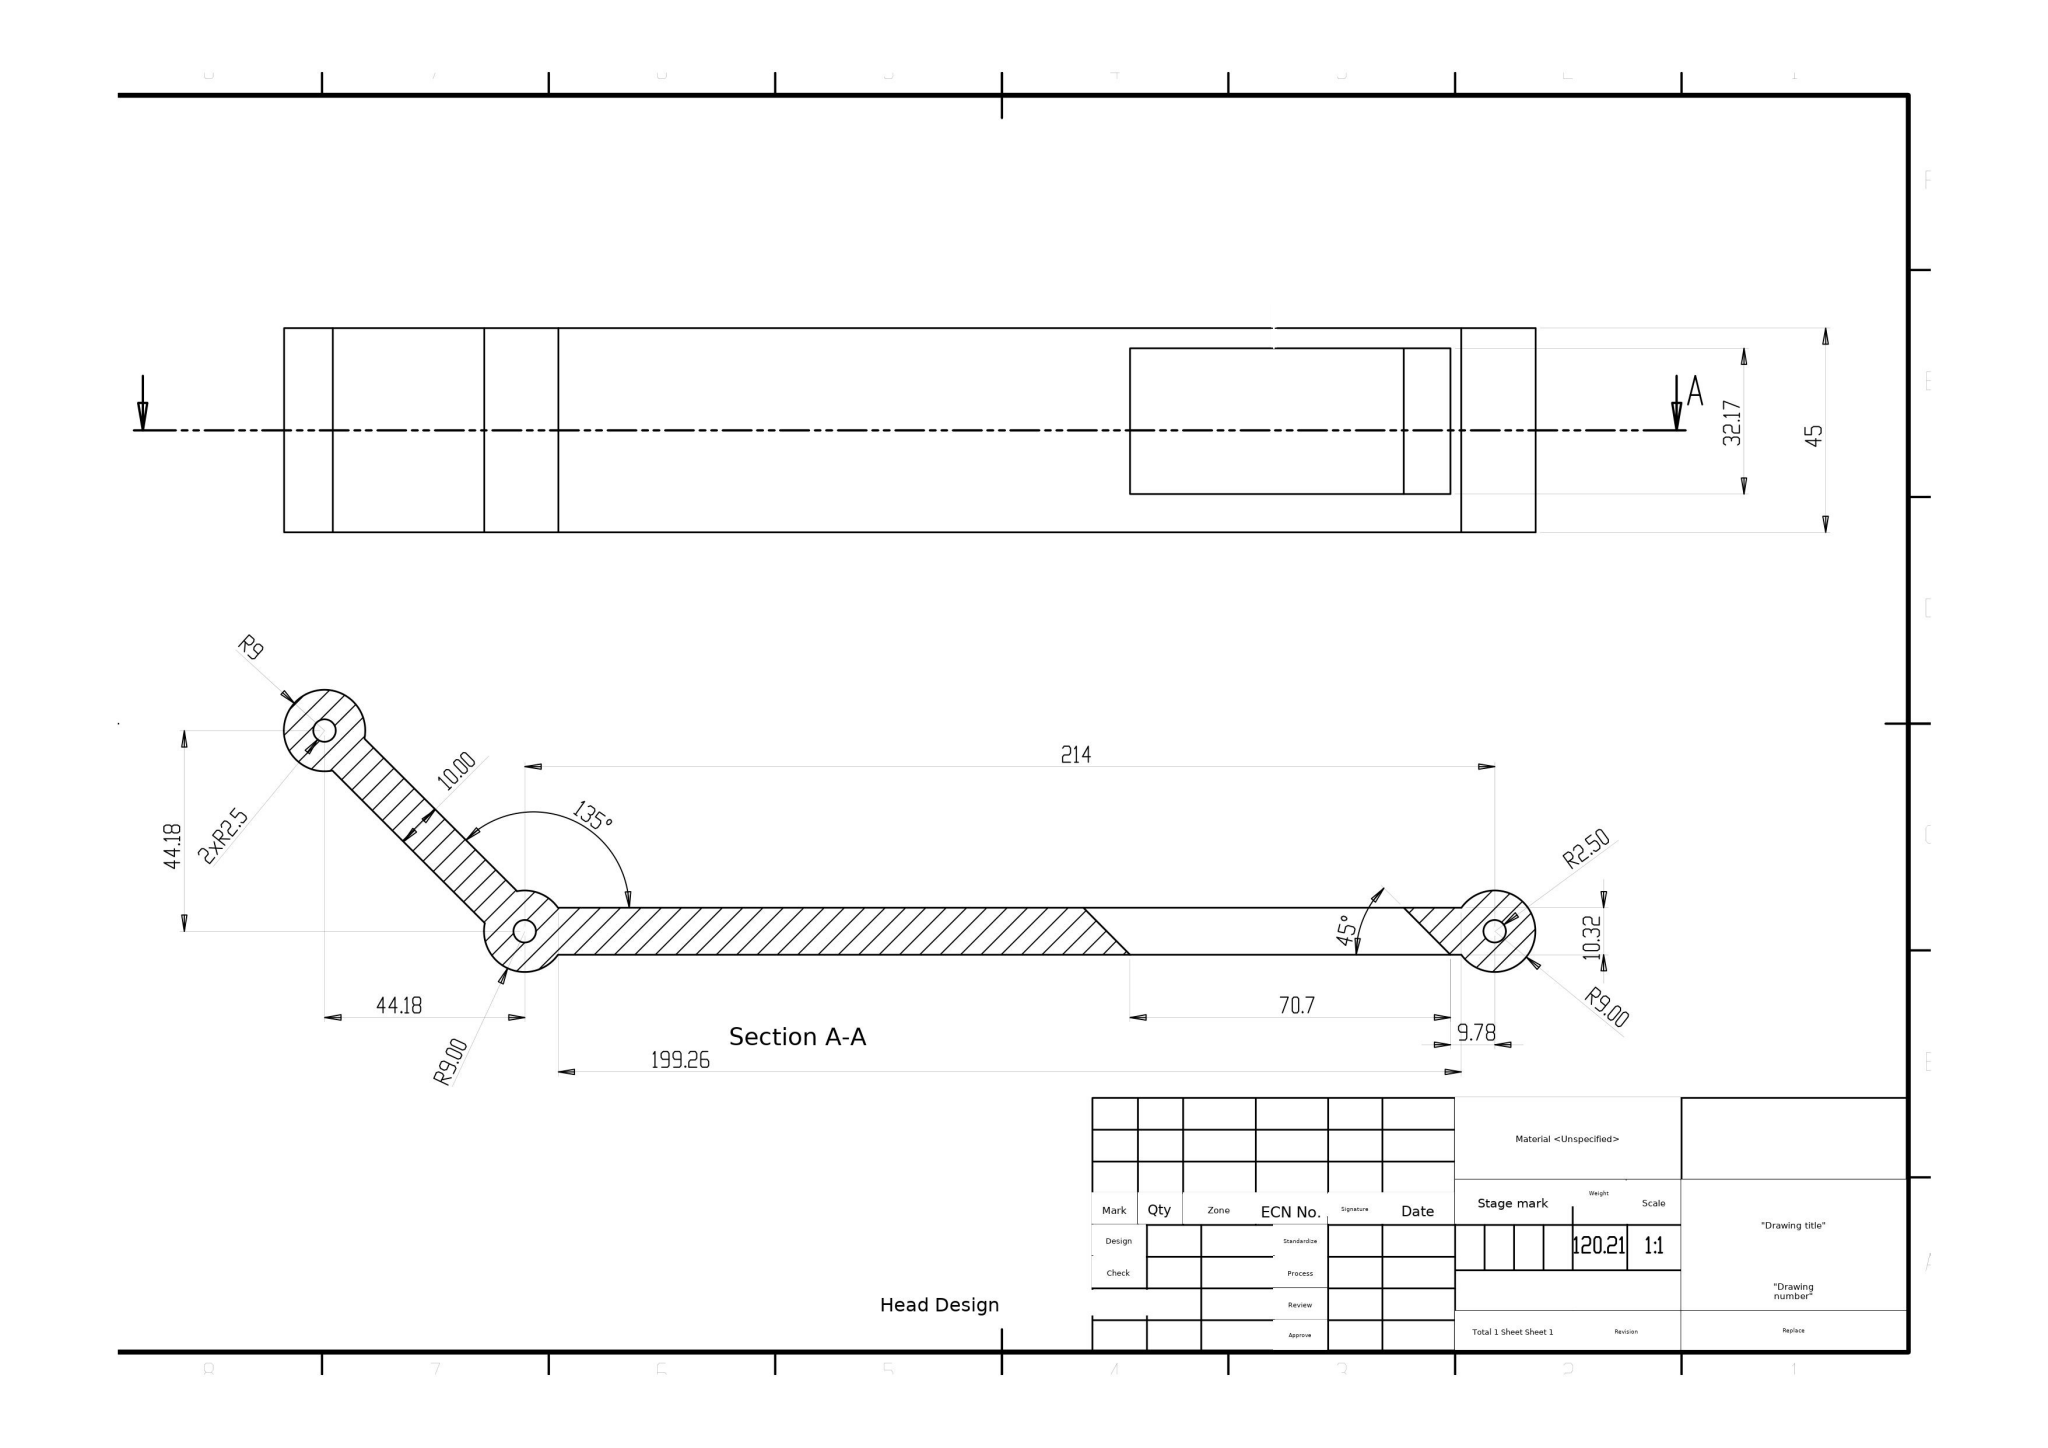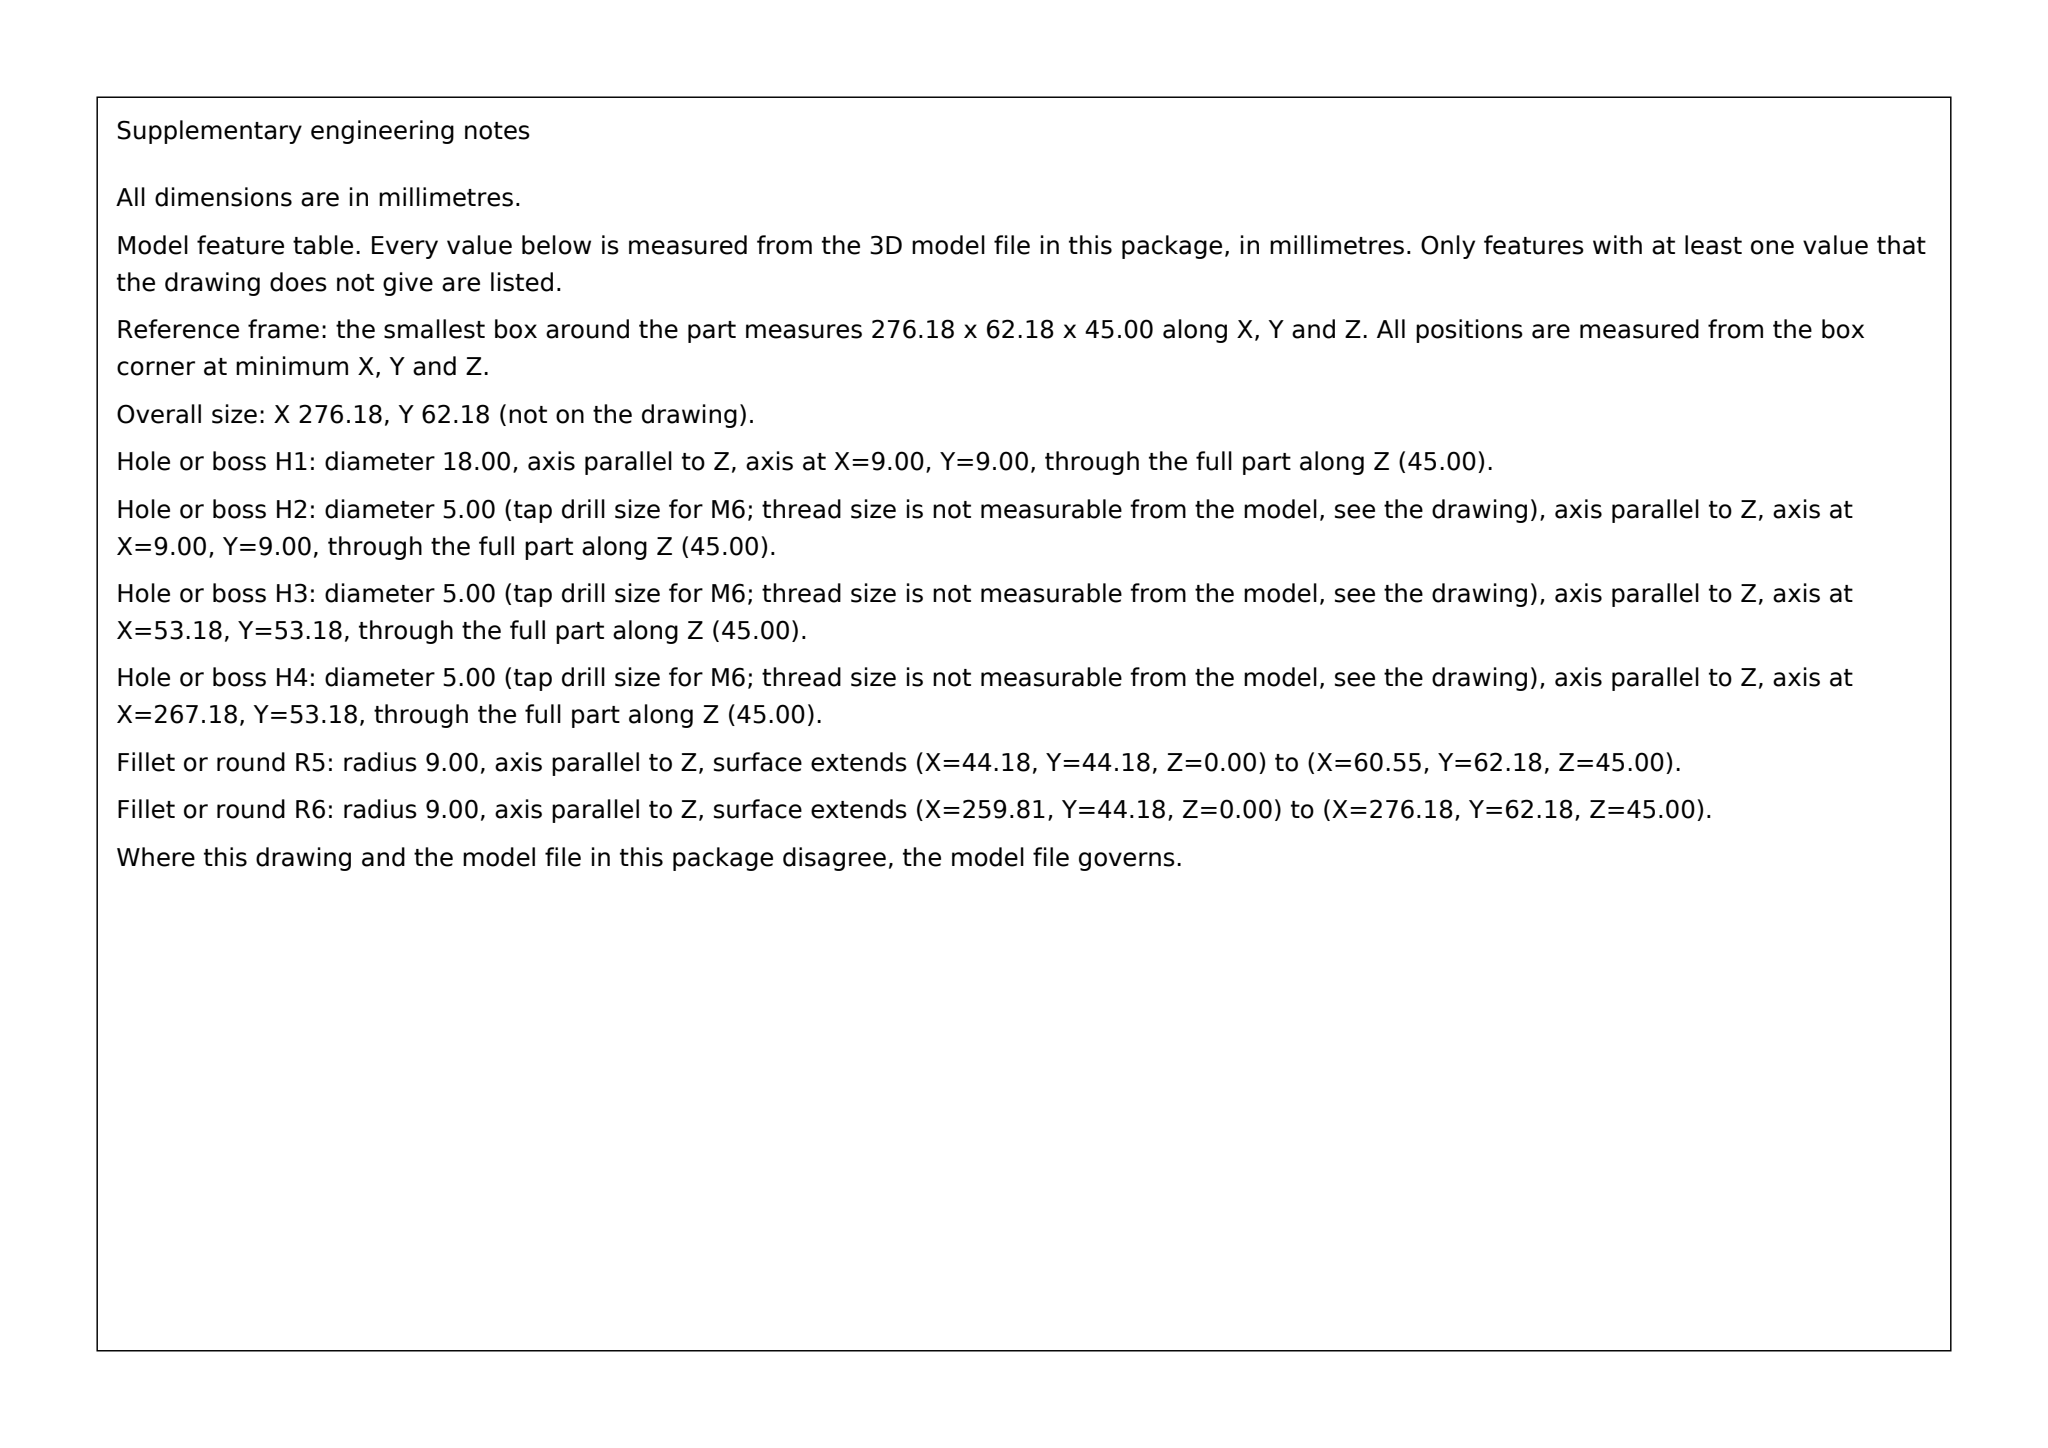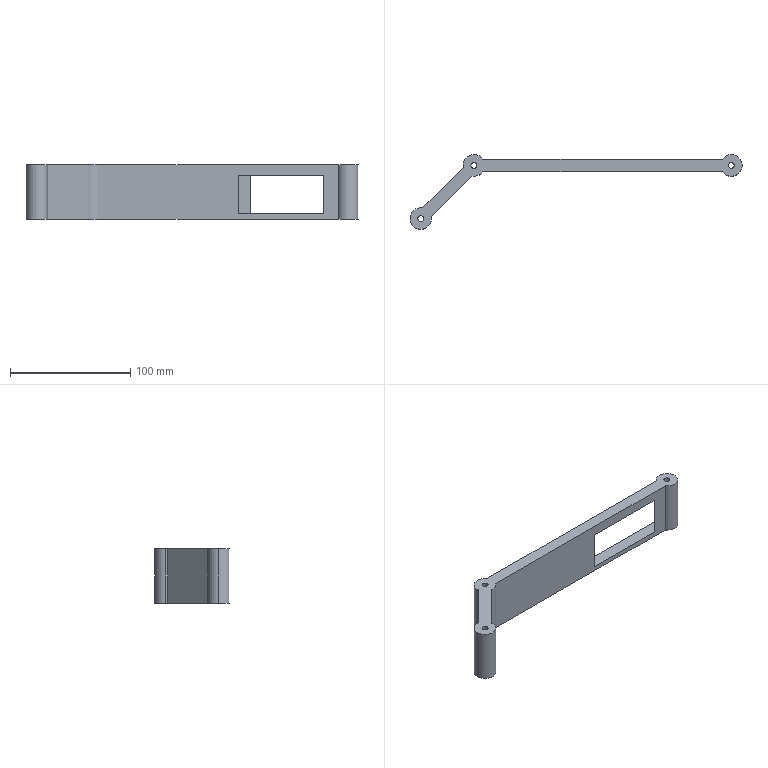Part | SolidWorks | mm | 1 solid | 23 faces | box 276.18 x 62.18 x 45 mm | volume 120214 mm3 | cylinder 13 | plane 10 | commonest cylinder face diameters 18 x7 5 x6
STEP:
#1=CARTESIAN_POINT('',(123.185,-5.162,36.594));
#2=VERTEX_POINT('',#1);
#3=CARTESIAN_POINT('',(133.509,5.162,36.594));
#4=VERTEX_POINT('',#3);
#5=CARTESIAN_POINT('',(10.993,-117.357,36.594));
#6=DIRECTION('',(0.7071,0.7071,0.));
#7=VECTOR('',#6,1000.);
#8=LINE('',#5,#7);
#9=EDGE_CURVE('',#2,#4,#8,.T.);
#10=ORIENTED_EDGE('',*,*,#9,.T.);
#11=CARTESIAN_POINT('',(204.219,5.162,36.594));
#12=VERTEX_POINT('',#11);
#13=CARTESIAN_POINT('',(-0.,5.162,36.594));
#14=DIRECTION('',(-1.,-0.,0.));
#15=VECTOR('',#14,1000.);
#16=LINE('',#13,#15);
#17=EDGE_CURVE('',#12,#4,#16,.T.);
#18=ORIENTED_EDGE('',*,*,#17,.F.);
#19=CARTESIAN_POINT('',(193.895,-5.162,36.594));
#20=VERTEX_POINT('',#19);
#21=CARTESIAN_POINT('',(46.349,-152.711,36.594));
#22=DIRECTION('',(0.7071,0.7071,0.));
#23=VECTOR('',#22,1000.);
#24=LINE('',#21,#23);
#25=EDGE_CURVE('',#20,#12,#24,.T.);
#26=ORIENTED_EDGE('',*,*,#25,.F.);
#27=CARTESIAN_POINT('',(-0.,-5.162,36.594));
#28=DIRECTION('',(1.,0.,-0.));
#29=VECTOR('',#28,1000.);
#30=LINE('',#27,#29);
#31=EDGE_CURVE('',#2,#20,#30,.T.);
#32=ORIENTED_EDGE('',*,*,#31,.F.);
#33=EDGE_LOOP('',(#10,#18,#26,#32));
#34=FACE_OUTER_BOUND('',#33,.T.);
#35=CARTESIAN_POINT('',(10.993,-117.357,36.594));
#36=DIRECTION('',(-0.,0.,-1.));
#37=DIRECTION('',(-1.,0.,0.));
#38=AXIS2_PLACEMENT_3D('',#35,#36,#37);
#39=PLANE('',#38);
#40=ADVANCED_FACE('',(#34),#39,.T.);
#41=ORIENTED_EDGE('',*,*,#25,.T.);
#42=CARTESIAN_POINT('',(204.219,5.162,4.421));
#43=VERTEX_POINT('',#42);
#44=CARTESIAN_POINT('',(204.219,5.162,45.));
#45=DIRECTION('',(0.,0.,1.));
#46=VECTOR('',#45,1000.);
#47=LINE('',#44,#46);
#48=EDGE_CURVE('',#43,#12,#47,.T.);
#49=ORIENTED_EDGE('',*,*,#48,.F.);
#50=CARTESIAN_POINT('',(193.895,-5.162,4.421));
#51=VERTEX_POINT('',#50);
#52=CARTESIAN_POINT('',(46.349,-152.711,4.421));
#53=DIRECTION('',(0.7071,0.7071,0.));
#54=VECTOR('',#53,1000.);
#55=LINE('',#52,#54);
#56=EDGE_CURVE('',#51,#43,#55,.T.);
#57=ORIENTED_EDGE('',*,*,#56,.F.);
#58=CARTESIAN_POINT('',(193.895,-5.162,45.));
#59=DIRECTION('',(-0.,0.,-1.));
#60=VECTOR('',#59,1000.);
#61=LINE('',#58,#60);
#62=EDGE_CURVE('',#20,#51,#61,.T.);
#63=ORIENTED_EDGE('',*,*,#62,.F.);
#64=EDGE_LOOP('',(#41,#49,#57,#63));
#65=FACE_OUTER_BOUND('',#64,.T.);
#66=CARTESIAN_POINT('',(46.349,-152.711,36.594));
#67=DIRECTION('',(-0.7071,0.7071,0.));
#68=DIRECTION('',(0.,0.,1.));
#69=AXIS2_PLACEMENT_3D('',#66,#67,#68);
#70=PLANE('',#69);
#71=ADVANCED_FACE('',(#65),#70,.T.);
#72=ORIENTED_EDGE('',*,*,#56,.T.);
#73=CARTESIAN_POINT('',(133.509,5.162,4.421));
#74=VERTEX_POINT('',#73);
#75=CARTESIAN_POINT('',(-0.,5.162,4.421));
#76=DIRECTION('',(1.,0.,-0.));
#77=VECTOR('',#76,1000.);
#78=LINE('',#75,#77);
#79=EDGE_CURVE('',#74,#43,#78,.T.);
#80=ORIENTED_EDGE('',*,*,#79,.F.);
#81=CARTESIAN_POINT('',(123.185,-5.162,4.421));
#82=VERTEX_POINT('',#81);
#83=CARTESIAN_POINT('',(10.993,-117.357,4.421));
#84=DIRECTION('',(0.7071,0.7071,0.));
#85=VECTOR('',#84,1000.);
#86=LINE('',#83,#85);
#87=EDGE_CURVE('',#82,#74,#86,.T.);
#88=ORIENTED_EDGE('',*,*,#87,.F.);
#89=CARTESIAN_POINT('',(-0.,-5.162,4.421));
#90=DIRECTION('',(-1.,0.,0.));
#91=VECTOR('',#90,1000.);
#92=LINE('',#89,#91);
#93=EDGE_CURVE('',#51,#82,#92,.T.);
#94=ORIENTED_EDGE('',*,*,#93,.F.);
#95=EDGE_LOOP('',(#72,#80,#88,#94));
#96=FACE_OUTER_BOUND('',#95,.T.);
#97=CARTESIAN_POINT('',(46.349,-152.711,4.421));
#98=DIRECTION('',(0.,-0.,1.));
#99=DIRECTION('',(0.,-1.,-0.));
#100=AXIS2_PLACEMENT_3D('',#97,#98,#99);
#101=PLANE('',#100);
#102=ADVANCED_FACE('',(#96),#101,.T.);
#103=ORIENTED_EDGE('',*,*,#87,.T.);
#104=CARTESIAN_POINT('',(133.509,5.162,45.));
#105=DIRECTION('',(-0.,-0.,-1.));
#106=VECTOR('',#105,1000.);
#107=LINE('',#104,#106);
#108=EDGE_CURVE('',#4,#74,#107,.T.);
#109=ORIENTED_EDGE('',*,*,#108,.F.);
#110=ORIENTED_EDGE('',*,*,#9,.F.);
#111=CARTESIAN_POINT('',(123.185,-5.162,45.));
#112=DIRECTION('',(0.,0.,1.));
#113=VECTOR('',#112,1000.);
#114=LINE('',#111,#113);
#115=EDGE_CURVE('',#82,#2,#114,.T.);
#116=ORIENTED_EDGE('',*,*,#115,.F.);
#117=EDGE_LOOP('',(#103,#109,#110,#116));
#118=FACE_OUTER_BOUND('',#117,.T.);
#119=CARTESIAN_POINT('',(10.993,-117.357,4.421));
#120=DIRECTION('',(0.7071,-0.7071,-0.));
#121=DIRECTION('',(0.,0.,-1.));
#122=AXIS2_PLACEMENT_3D('',#119,#120,#121);
#123=PLANE('',#122);
#124=ADVANCED_FACE('',(#118),#123,.T.);
#125=CARTESIAN_POINT('',(-46.682,-44.182,0.));
#126=VERTEX_POINT('',#125);
#127=CARTESIAN_POINT('',(-41.682,-44.182,0.));
#128=VERTEX_POINT('',#127);
#129=CARTESIAN_POINT('',(-44.182,-44.182,0.));
#130=DIRECTION('',(0.,0.,1.));
#131=DIRECTION('',(1.,0.,0.));
#132=AXIS2_PLACEMENT_3D('',#129,#130,#131);
#133=CIRCLE('',#132,2.5);
#134=EDGE_CURVE('',#126,#128,#133,.T.);
#135=ORIENTED_EDGE('',*,*,#134,.T.);
#136=CARTESIAN_POINT('',(-44.182,-44.182,0.));
#137=DIRECTION('',(0.,0.,1.));
#138=DIRECTION('',(1.,0.,0.));
#139=AXIS2_PLACEMENT_3D('',#136,#137,#138);
#140=CIRCLE('',#139,2.5);
#141=EDGE_CURVE('',#128,#126,#140,.T.);
#142=ORIENTED_EDGE('',*,*,#141,.T.);
#143=EDGE_LOOP('',(#135,#142));
#144=FACE_BOUND('',#143,.T.);
#145=CARTESIAN_POINT('',(211.5,0.,0.));
#146=VERTEX_POINT('',#145);
#147=CARTESIAN_POINT('',(216.5,0.,0.));
#148=VERTEX_POINT('',#147);
#149=CARTESIAN_POINT('',(214.,0.,0.));
#150=DIRECTION('',(0.,0.,1.));
#151=DIRECTION('',(1.,0.,0.));
#152=AXIS2_PLACEMENT_3D('',#149,#150,#151);
#153=CIRCLE('',#152,2.5);
#154=EDGE_CURVE('',#146,#148,#153,.T.);
#155=ORIENTED_EDGE('',*,*,#154,.T.);
#156=CARTESIAN_POINT('',(214.,0.,0.));
#157=DIRECTION('',(0.,0.,1.));
#158=DIRECTION('',(1.,0.,0.));
#159=AXIS2_PLACEMENT_3D('',#156,#157,#158);
#160=CIRCLE('',#159,2.5);
#161=EDGE_CURVE('',#148,#146,#160,.T.);
#162=ORIENTED_EDGE('',*,*,#161,.T.);
#163=EDGE_LOOP('',(#155,#162));
#164=FACE_BOUND('',#163,.T.);
#165=CARTESIAN_POINT('',(-2.5,0.,0.));
#166=VERTEX_POINT('',#165);
#167=CARTESIAN_POINT('',(2.5,0.,0.));
#168=VERTEX_POINT('',#167);
#169=CARTESIAN_POINT('',(0.,0.,0.));
#170=DIRECTION('',(0.,0.,1.));
#171=DIRECTION('',(1.,0.,0.));
#172=AXIS2_PLACEMENT_3D('',#169,#170,#171);
#173=CIRCLE('',#172,2.5);
#174=EDGE_CURVE('',#166,#168,#173,.T.);
#175=ORIENTED_EDGE('',*,*,#174,.T.);
#176=CARTESIAN_POINT('',(0.,0.,0.));
#177=DIRECTION('',(0.,0.,1.));
#178=DIRECTION('',(1.,0.,0.));
#179=AXIS2_PLACEMENT_3D('',#176,#177,#178);
#180=CIRCLE('',#179,2.5);
#181=EDGE_CURVE('',#168,#166,#180,.T.);
#182=ORIENTED_EDGE('',*,*,#181,.T.);
#183=EDGE_LOOP('',(#175,#182));
#184=FACE_BOUND('',#183,.T.);
#185=CARTESIAN_POINT('',(7.372,5.162,0.));
#186=VERTEX_POINT('',#185);
#187=CARTESIAN_POINT('',(-9.,0.,0.));
#188=VERTEX_POINT('',#187);
#189=CARTESIAN_POINT('',(0.,0.,0.));
#190=DIRECTION('',(0.,0.,1.));
#191=DIRECTION('',(1.,0.,0.));
#192=AXIS2_PLACEMENT_3D('',#189,#190,#191);
#193=CIRCLE('',#192,9.);
#194=EDGE_CURVE('',#186,#188,#193,.T.);
#195=ORIENTED_EDGE('',*,*,#194,.F.);
#196=CARTESIAN_POINT('',(206.628,5.162,0.));
#197=VERTEX_POINT('',#196);
#198=CARTESIAN_POINT('',(-0.,5.162,0.));
#199=DIRECTION('',(1.,0.,0.));
#200=VECTOR('',#199,1000.);
#201=LINE('',#198,#200);
#202=EDGE_CURVE('',#186,#197,#201,.T.);
#203=ORIENTED_EDGE('',*,*,#202,.T.);
#204=CARTESIAN_POINT('',(206.628,-5.162,0.));
#205=VERTEX_POINT('',#204);
#206=CARTESIAN_POINT('',(214.,0.,0.));
#207=DIRECTION('',(0.,0.,1.));
#208=DIRECTION('',(1.,0.,0.));
#209=AXIS2_PLACEMENT_3D('',#206,#207,#208);
#210=CIRCLE('',#209,9.);
#211=EDGE_CURVE('',#205,#197,#210,.T.);
#212=ORIENTED_EDGE('',*,*,#211,.F.);
#213=CARTESIAN_POINT('',(7.372,-5.162,0.));
#214=VERTEX_POINT('',#213);
#215=CARTESIAN_POINT('',(0.,-5.162,0.));
#216=DIRECTION('',(-1.,0.,0.));
#217=VECTOR('',#216,1000.);
#218=LINE('',#215,#217);
#219=EDGE_CURVE('',#205,#214,#218,.T.);
#220=ORIENTED_EDGE('',*,*,#219,.T.);
#221=CARTESIAN_POINT('',(-1.756,-8.827,0.));
#222=VERTEX_POINT('',#221);
#223=CARTESIAN_POINT('',(0.,0.,0.));
#224=DIRECTION('',(0.,0.,1.));
#225=DIRECTION('',(1.,0.,0.));
#226=AXIS2_PLACEMENT_3D('',#223,#224,#225);
#227=CIRCLE('',#226,9.);
#228=EDGE_CURVE('',#222,#214,#227,.T.);
#229=ORIENTED_EDGE('',*,*,#228,.F.);
#230=CARTESIAN_POINT('',(-35.355,-42.426,0.));
#231=VERTEX_POINT('',#230);
#232=CARTESIAN_POINT('',(3.536,-3.536,0.));
#233=DIRECTION('',(-0.7071,-0.7071,0.));
#234=VECTOR('',#233,1000.);
#235=LINE('',#232,#234);
#236=EDGE_CURVE('',#222,#231,#235,.T.);
#237=ORIENTED_EDGE('',*,*,#236,.T.);
#238=CARTESIAN_POINT('',(-35.182,-44.182,0.));
#239=VERTEX_POINT('',#238);
#240=CARTESIAN_POINT('',(-44.182,-44.182,0.));
#241=DIRECTION('',(0.,0.,1.));
#242=DIRECTION('',(1.,0.,0.));
#243=AXIS2_PLACEMENT_3D('',#240,#241,#242);
#244=CIRCLE('',#243,9.);
#245=EDGE_CURVE('',#239,#231,#244,.T.);
#246=ORIENTED_EDGE('',*,*,#245,.F.);
#247=CARTESIAN_POINT('',(-53.182,-44.182,0.));
#248=VERTEX_POINT('',#247);
#249=CARTESIAN_POINT('',(-44.182,-44.182,0.));
#250=DIRECTION('',(0.,0.,1.));
#251=DIRECTION('',(1.,0.,0.));
#252=AXIS2_PLACEMENT_3D('',#249,#250,#251);
#253=CIRCLE('',#252,9.);
#254=EDGE_CURVE('',#248,#239,#253,.T.);
#255=ORIENTED_EDGE('',*,*,#254,.F.);
#256=CARTESIAN_POINT('',(-42.426,-35.355,0.));
#257=VERTEX_POINT('',#256);
#258=CARTESIAN_POINT('',(-44.182,-44.182,0.));
#259=DIRECTION('',(0.,0.,1.));
#260=DIRECTION('',(1.,0.,0.));
#261=AXIS2_PLACEMENT_3D('',#258,#259,#260);
#262=CIRCLE('',#261,9.);
#263=EDGE_CURVE('',#257,#248,#262,.T.);
#264=ORIENTED_EDGE('',*,*,#263,.F.);
#265=CARTESIAN_POINT('',(-8.827,-1.756,0.));
#266=VERTEX_POINT('',#265);
#267=CARTESIAN_POINT('',(-3.536,3.536,0.));
#268=DIRECTION('',(-0.7071,-0.7071,0.));
#269=VECTOR('',#268,1000.);
#270=LINE('',#267,#269);
#271=EDGE_CURVE('',#266,#257,#270,.T.);
#272=ORIENTED_EDGE('',*,*,#271,.F.);
#273=CARTESIAN_POINT('',(0.,0.,0.));
#274=DIRECTION('',(0.,0.,1.));
#275=DIRECTION('',(1.,0.,0.));
#276=AXIS2_PLACEMENT_3D('',#273,#274,#275);
#277=CIRCLE('',#276,9.);
#278=EDGE_CURVE('',#188,#266,#277,.T.);
#279=ORIENTED_EDGE('',*,*,#278,.F.);
#280=EDGE_LOOP('',(#195,#203,#212,#220,#229,#237,#246,#255,#264,#272,#279));
#281=FACE_OUTER_BOUND('',#280,.T.);
#282=CARTESIAN_POINT('',(0.,0.,0.));
#283=DIRECTION('',(0.,0.,1.));
#284=DIRECTION('',(1.,0.,0.));
#285=AXIS2_PLACEMENT_3D('',#282,#283,#284);
#286=PLANE('',#285);
#287=ADVANCED_FACE('',(#144,#164,#184,#281),#286,.F.);
#288=CARTESIAN_POINT('',(-46.682,-44.182,45.));
#289=VERTEX_POINT('',#288);
#290=CARTESIAN_POINT('',(-41.682,-44.182,45.));
#291=VERTEX_POINT('',#290);
#292=CARTESIAN_POINT('',(-44.182,-44.182,45.));
#293=DIRECTION('',(0.,0.,1.));
#294=DIRECTION('',(1.,0.,0.));
#295=AXIS2_PLACEMENT_3D('',#292,#293,#294);
#296=CIRCLE('',#295,2.5);
#297=EDGE_CURVE('',#289,#291,#296,.T.);
#298=ORIENTED_EDGE('',*,*,#297,.F.);
#299=CARTESIAN_POINT('',(-44.182,-44.182,45.));
#300=DIRECTION('',(0.,0.,1.));
#301=DIRECTION('',(1.,0.,0.));
#302=AXIS2_PLACEMENT_3D('',#299,#300,#301);
#303=CIRCLE('',#302,2.5);
#304=EDGE_CURVE('',#291,#289,#303,.T.);
#305=ORIENTED_EDGE('',*,*,#304,.F.);
#306=EDGE_LOOP('',(#298,#305));
#307=FACE_BOUND('',#306,.T.);
#308=CARTESIAN_POINT('',(211.5,0.,45.));
#309=VERTEX_POINT('',#308);
#310=CARTESIAN_POINT('',(216.5,0.,45.));
#311=VERTEX_POINT('',#310);
#312=CARTESIAN_POINT('',(214.,0.,45.));
#313=DIRECTION('',(0.,0.,1.));
#314=DIRECTION('',(1.,0.,0.));
#315=AXIS2_PLACEMENT_3D('',#312,#313,#314);
#316=CIRCLE('',#315,2.5);
#317=EDGE_CURVE('',#309,#311,#316,.T.);
#318=ORIENTED_EDGE('',*,*,#317,.F.);
#319=CARTESIAN_POINT('',(214.,0.,45.));
#320=DIRECTION('',(0.,0.,1.));
#321=DIRECTION('',(1.,0.,0.));
#322=AXIS2_PLACEMENT_3D('',#319,#320,#321);
#323=CIRCLE('',#322,2.5);
#324=EDGE_CURVE('',#311,#309,#323,.T.);
#325=ORIENTED_EDGE('',*,*,#324,.F.);
#326=EDGE_LOOP('',(#318,#325));
#327=FACE_BOUND('',#326,.T.);
#328=CARTESIAN_POINT('',(-2.5,0.,45.));
#329=VERTEX_POINT('',#328);
#330=CARTESIAN_POINT('',(2.5,0.,45.));
#331=VERTEX_POINT('',#330);
#332=CARTESIAN_POINT('',(0.,0.,45.));
#333=DIRECTION('',(0.,0.,1.));
#334=DIRECTION('',(1.,0.,0.));
#335=AXIS2_PLACEMENT_3D('',#332,#333,#334);
#336=CIRCLE('',#335,2.5);
#337=EDGE_CURVE('',#329,#331,#336,.T.);
#338=ORIENTED_EDGE('',*,*,#337,.F.);
#339=CARTESIAN_POINT('',(0.,0.,45.));
#340=DIRECTION('',(0.,0.,1.));
#341=DIRECTION('',(1.,0.,0.));
#342=AXIS2_PLACEMENT_3D('',#339,#340,#341);
#343=CIRCLE('',#342,2.5);
#344=EDGE_CURVE('',#331,#329,#343,.T.);
#345=ORIENTED_EDGE('',*,*,#344,.F.);
#346=EDGE_LOOP('',(#338,#345));
#347=FACE_BOUND('',#346,.T.);
#348=CARTESIAN_POINT('',(7.372,5.162,45.));
#349=VERTEX_POINT('',#348);
#350=CARTESIAN_POINT('',(-9.,0.,45.));
#351=VERTEX_POINT('',#350);
#352=CARTESIAN_POINT('',(0.,0.,45.));
#353=DIRECTION('',(0.,0.,1.));
#354=DIRECTION('',(1.,0.,0.));
#355=AXIS2_PLACEMENT_3D('',#352,#353,#354);
#356=CIRCLE('',#355,9.);
#357=EDGE_CURVE('',#349,#351,#356,.T.);
#358=ORIENTED_EDGE('',*,*,#357,.T.);
#359=CARTESIAN_POINT('',(-8.827,-1.756,45.));
#360=VERTEX_POINT('',#359);
#361=CARTESIAN_POINT('',(0.,0.,45.));
#362=DIRECTION('',(0.,0.,1.));
#363=DIRECTION('',(1.,0.,0.));
#364=AXIS2_PLACEMENT_3D('',#361,#362,#363);
#365=CIRCLE('',#364,9.);
#366=EDGE_CURVE('',#351,#360,#365,.T.);
#367=ORIENTED_EDGE('',*,*,#366,.T.);
#368=CARTESIAN_POINT('',(-42.426,-35.355,45.));
#369=VERTEX_POINT('',#368);
#370=CARTESIAN_POINT('',(-3.536,3.536,45.));
#371=DIRECTION('',(-0.7071,-0.7071,0.));
#372=VECTOR('',#371,1000.);
#373=LINE('',#370,#372);
#374=EDGE_CURVE('',#360,#369,#373,.T.);
#375=ORIENTED_EDGE('',*,*,#374,.T.);
#376=CARTESIAN_POINT('',(-53.182,-44.182,45.));
#377=VERTEX_POINT('',#376);
#378=CARTESIAN_POINT('',(-44.182,-44.182,45.));
#379=DIRECTION('',(0.,0.,1.));
#380=DIRECTION('',(1.,0.,0.));
#381=AXIS2_PLACEMENT_3D('',#378,#379,#380);
#382=CIRCLE('',#381,9.);
#383=EDGE_CURVE('',#369,#377,#382,.T.);
#384=ORIENTED_EDGE('',*,*,#383,.T.);
#385=CARTESIAN_POINT('',(-35.182,-44.182,45.));
#386=VERTEX_POINT('',#385);
#387=CARTESIAN_POINT('',(-44.182,-44.182,45.));
#388=DIRECTION('',(0.,0.,1.));
#389=DIRECTION('',(1.,0.,0.));
#390=AXIS2_PLACEMENT_3D('',#387,#388,#389);
#391=CIRCLE('',#390,9.);
#392=EDGE_CURVE('',#377,#386,#391,.T.);
#393=ORIENTED_EDGE('',*,*,#392,.T.);
#394=CARTESIAN_POINT('',(-35.355,-42.426,45.));
#395=VERTEX_POINT('',#394);
#396=CARTESIAN_POINT('',(-44.182,-44.182,45.));
#397=DIRECTION('',(0.,0.,1.));
#398=DIRECTION('',(1.,0.,0.));
#399=AXIS2_PLACEMENT_3D('',#396,#397,#398);
#400=CIRCLE('',#399,9.);
#401=EDGE_CURVE('',#386,#395,#400,.T.);
#402=ORIENTED_EDGE('',*,*,#401,.T.);
#403=CARTESIAN_POINT('',(-1.756,-8.827,45.));
#404=VERTEX_POINT('',#403);
#405=CARTESIAN_POINT('',(3.536,-3.536,45.));
#406=DIRECTION('',(-0.7071,-0.7071,0.));
#407=VECTOR('',#406,1000.);
#408=LINE('',#405,#407);
#409=EDGE_CURVE('',#404,#395,#408,.T.);
#410=ORIENTED_EDGE('',*,*,#409,.F.);
#411=CARTESIAN_POINT('',(7.372,-5.162,45.));
#412=VERTEX_POINT('',#411);
#413=CARTESIAN_POINT('',(0.,0.,45.));
#414=DIRECTION('',(0.,0.,1.));
#415=DIRECTION('',(1.,0.,0.));
#416=AXIS2_PLACEMENT_3D('',#413,#414,#415);
#417=CIRCLE('',#416,9.);
#418=EDGE_CURVE('',#404,#412,#417,.T.);
#419=ORIENTED_EDGE('',*,*,#418,.T.);
#420=CARTESIAN_POINT('',(206.628,-5.162,45.));
#421=VERTEX_POINT('',#420);
#422=CARTESIAN_POINT('',(0.,-5.162,45.));
#423=DIRECTION('',(-1.,0.,0.));
#424=VECTOR('',#423,1000.);
#425=LINE('',#422,#424);
#426=EDGE_CURVE('',#421,#412,#425,.T.);
#427=ORIENTED_EDGE('',*,*,#426,.F.);
#428=CARTESIAN_POINT('',(206.628,5.162,45.));
#429=VERTEX_POINT('',#428);
#430=CARTESIAN_POINT('',(214.,0.,45.));
#431=DIRECTION('',(0.,0.,1.));
#432=DIRECTION('',(1.,0.,0.));
#433=AXIS2_PLACEMENT_3D('',#430,#431,#432);
#434=CIRCLE('',#433,9.);
#435=EDGE_CURVE('',#421,#429,#434,.T.);
#436=ORIENTED_EDGE('',*,*,#435,.T.);
#437=CARTESIAN_POINT('',(-0.,5.162,45.));
#438=DIRECTION('',(1.,0.,0.));
#439=VECTOR('',#438,1000.);
#440=LINE('',#437,#439);
#441=EDGE_CURVE('',#349,#429,#440,.T.);
#442=ORIENTED_EDGE('',*,*,#441,.F.);
#443=EDGE_LOOP('',(#358,#367,#375,#384,#393,#402,#410,#419,#427,#436,#442));
#444=FACE_OUTER_BOUND('',#443,.T.);
#445=CARTESIAN_POINT('',(0.,0.,45.));
#446=DIRECTION('',(0.,0.,1.));
#447=DIRECTION('',(1.,0.,0.));
#448=AXIS2_PLACEMENT_3D('',#445,#446,#447);
#449=PLANE('',#448);
#450=ADVANCED_FACE('',(#307,#327,#347,#444),#449,.T.);
#451=CARTESIAN_POINT('',(-41.682,-44.182,45.));
#452=DIRECTION('',(0.,0.,-1.));
#453=VECTOR('',#452,1000.);
#454=LINE('',#451,#453);
#455=EDGE_CURVE('',#291,#128,#454,.T.);
#456=ORIENTED_EDGE('',*,*,#455,.F.);
#457=ORIENTED_EDGE('',*,*,#304,.T.);
#458=CARTESIAN_POINT('',(-46.682,-44.182,45.));
#459=DIRECTION('',(0.,0.,-1.));
#460=VECTOR('',#459,1000.);
#461=LINE('',#458,#460);
#462=EDGE_CURVE('',#289,#126,#461,.T.);
#463=ORIENTED_EDGE('',*,*,#462,.T.);
#464=ORIENTED_EDGE('',*,*,#141,.F.);
#465=EDGE_LOOP('',(#456,#457,#463,#464));
#466=FACE_OUTER_BOUND('',#465,.T.);
#467=CARTESIAN_POINT('',(-44.182,-44.182,45.));
#468=DIRECTION('',(0.,0.,-1.));
#469=DIRECTION('',(-1.,0.,0.));
#470=AXIS2_PLACEMENT_3D('',#467,#468,#469);
#471=CYLINDRICAL_SURFACE('',#470,2.5);
#472=ADVANCED_FACE('',(#466),#471,.F.);
#473=CARTESIAN_POINT('',(2.5,0.,45.));
#474=DIRECTION('',(0.,0.,-1.));
#475=VECTOR('',#474,1000.);
#476=LINE('',#473,#475);
#477=EDGE_CURVE('',#331,#168,#476,.T.);
#478=ORIENTED_EDGE('',*,*,#477,.F.);
#479=ORIENTED_EDGE('',*,*,#344,.T.);
#480=CARTESIAN_POINT('',(-2.5,0.,45.));
#481=DIRECTION('',(0.,0.,-1.));
#482=VECTOR('',#481,1000.);
#483=LINE('',#480,#482);
#484=EDGE_CURVE('',#329,#166,#483,.T.);
#485=ORIENTED_EDGE('',*,*,#484,.T.);
#486=ORIENTED_EDGE('',*,*,#181,.F.);
#487=EDGE_LOOP('',(#478,#479,#485,#486));
#488=FACE_OUTER_BOUND('',#487,.T.);
#489=CARTESIAN_POINT('',(0.,0.,45.));
#490=DIRECTION('',(0.,0.,-1.));
#491=DIRECTION('',(-1.,0.,0.));
#492=AXIS2_PLACEMENT_3D('',#489,#490,#491);
#493=CYLINDRICAL_SURFACE('',#492,2.5);
#494=ADVANCED_FACE('',(#488),#493,.F.);
#495=CARTESIAN_POINT('',(216.5,0.,45.));
#496=DIRECTION('',(0.,0.,-1.));
#497=VECTOR('',#496,1000.);
#498=LINE('',#495,#497);
#499=EDGE_CURVE('',#311,#148,#498,.T.);
#500=ORIENTED_EDGE('',*,*,#499,.F.);
#501=ORIENTED_EDGE('',*,*,#324,.T.);
#502=CARTESIAN_POINT('',(211.5,0.,45.));
#503=DIRECTION('',(0.,0.,-1.));
#504=VECTOR('',#503,1000.);
#505=LINE('',#502,#504);
#506=EDGE_CURVE('',#309,#146,#505,.T.);
#507=ORIENTED_EDGE('',*,*,#506,.T.);
#508=ORIENTED_EDGE('',*,*,#161,.F.);
#509=EDGE_LOOP('',(#500,#501,#507,#508));
#510=FACE_OUTER_BOUND('',#509,.T.);
#511=CARTESIAN_POINT('',(214.,0.,45.));
#512=DIRECTION('',(0.,0.,-1.));
#513=DIRECTION('',(-1.,0.,0.));
#514=AXIS2_PLACEMENT_3D('',#511,#512,#513);
#515=CYLINDRICAL_SURFACE('',#514,2.5);
#516=ADVANCED_FACE('',(#510),#515,.F.);
#517=ORIENTED_EDGE('',*,*,#211,.T.);
#518=CARTESIAN_POINT('',(206.628,5.162,45.));
#519=DIRECTION('',(0.,0.,-1.));
#520=VECTOR('',#519,1000.);
#521=LINE('',#518,#520);
#522=EDGE_CURVE('',#429,#197,#521,.T.);
#523=ORIENTED_EDGE('',*,*,#522,.F.);
#524=ORIENTED_EDGE('',*,*,#435,.F.);
#525=CARTESIAN_POINT('',(206.628,-5.162,45.));
#526=DIRECTION('',(0.,0.,-1.));
#527=VECTOR('',#526,1000.);
#528=LINE('',#525,#527);
#529=EDGE_CURVE('',#421,#205,#528,.T.);
#530=ORIENTED_EDGE('',*,*,#529,.T.);
#531=EDGE_LOOP('',(#517,#523,#524,#530));
#532=FACE_OUTER_BOUND('',#531,.T.);
#533=CARTESIAN_POINT('',(214.,0.,45.));
#534=DIRECTION('',(0.,0.,-1.));
#535=DIRECTION('',(-1.,0.,0.));
#536=AXIS2_PLACEMENT_3D('',#533,#534,#535);
#537=CYLINDRICAL_SURFACE('',#536,9.);
#538=ADVANCED_FACE('',(#532),#537,.T.);
#539=ORIENTED_EDGE('',*,*,#228,.T.);
#540=CARTESIAN_POINT('',(7.372,-5.162,45.));
#541=DIRECTION('',(0.,0.,-1.));
#542=VECTOR('',#541,1000.);
#543=LINE('',#540,#542);
#544=EDGE_CURVE('',#412,#214,#543,.T.);
#545=ORIENTED_EDGE('',*,*,#544,.F.);
#546=ORIENTED_EDGE('',*,*,#418,.F.);
#547=CARTESIAN_POINT('',(-1.756,-8.827,45.));
#548=DIRECTION('',(0.,0.,-1.));
#549=VECTOR('',#548,1000.);
#550=LINE('',#547,#549);
#551=EDGE_CURVE('',#404,#222,#550,.T.);
#552=ORIENTED_EDGE('',*,*,#551,.T.);
#553=EDGE_LOOP('',(#539,#545,#546,#552));
#554=FACE_OUTER_BOUND('',#553,.T.);
#555=CARTESIAN_POINT('',(0.,0.,45.));
#556=DIRECTION('',(0.,0.,-1.));
#557=DIRECTION('',(-1.,0.,0.));
#558=AXIS2_PLACEMENT_3D('',#555,#556,#557);
#559=CYLINDRICAL_SURFACE('',#558,9.);
#560=ADVANCED_FACE('',(#554),#559,.T.);
#561=ORIENTED_EDGE('',*,*,#236,.F.);
#562=ORIENTED_EDGE('',*,*,#551,.F.);
#563=ORIENTED_EDGE('',*,*,#409,.T.);
#564=CARTESIAN_POINT('',(-35.355,-42.426,45.));
#565=DIRECTION('',(0.,0.,-1.));
#566=VECTOR('',#565,1000.);
#567=LINE('',#564,#566);
#568=EDGE_CURVE('',#395,#231,#567,.T.);
#569=ORIENTED_EDGE('',*,*,#568,.T.);
#570=EDGE_LOOP('',(#561,#562,#563,#569));
#571=FACE_OUTER_BOUND('',#570,.T.);
#572=CARTESIAN_POINT('',(3.536,-3.536,45.));
#573=DIRECTION('',(0.7071,-0.7071,0.));
#574=DIRECTION('',(0.,0.,-1.));
#575=AXIS2_PLACEMENT_3D('',#572,#573,#574);
#576=PLANE('',#575);
#577=ADVANCED_FACE('',(#571),#576,.T.);
#578=CARTESIAN_POINT('',(-53.182,-44.182,45.));
#579=DIRECTION('',(0.,0.,-1.));
#580=VECTOR('',#579,1000.);
#581=LINE('',#578,#580);
#582=EDGE_CURVE('',#377,#248,#581,.T.);
#583=ORIENTED_EDGE('',*,*,#582,.F.);
#584=ORIENTED_EDGE('',*,*,#383,.F.);
#585=CARTESIAN_POINT('',(-42.426,-35.355,45.));
#586=DIRECTION('',(0.,0.,-1.));
#587=VECTOR('',#586,1000.);
#588=LINE('',#585,#587);
#589=EDGE_CURVE('',#369,#257,#588,.T.);
#590=ORIENTED_EDGE('',*,*,#589,.T.);
#591=ORIENTED_EDGE('',*,*,#263,.T.);
#592=EDGE_LOOP('',(#583,#584,#590,#591));
#593=FACE_OUTER_BOUND('',#592,.T.);
#594=CARTESIAN_POINT('',(-44.182,-44.182,45.));
#595=DIRECTION('',(0.,0.,-1.));
#596=DIRECTION('',(-1.,0.,0.));
#597=AXIS2_PLACEMENT_3D('',#594,#595,#596);
#598=CYLINDRICAL_SURFACE('',#597,9.);
#599=ADVANCED_FACE('',(#593),#598,.T.);
#600=ORIENTED_EDGE('',*,*,#271,.T.);
#601=ORIENTED_EDGE('',*,*,#589,.F.);
#602=ORIENTED_EDGE('',*,*,#374,.F.);
#603=CARTESIAN_POINT('',(-8.827,-1.756,45.));
#604=DIRECTION('',(0.,0.,-1.));
#605=VECTOR('',#604,1000.);
#606=LINE('',#603,#605);
#607=EDGE_CURVE('',#360,#266,#606,.T.);
#608=ORIENTED_EDGE('',*,*,#607,.T.);
#609=EDGE_LOOP('',(#600,#601,#602,#608));
#610=FACE_OUTER_BOUND('',#609,.T.);
#611=CARTESIAN_POINT('',(-3.536,3.536,45.));
#612=DIRECTION('',(0.7071,-0.7071,0.));
#613=DIRECTION('',(0.,0.,-1.));
#614=AXIS2_PLACEMENT_3D('',#611,#612,#613);
#615=PLANE('',#614);
#616=ADVANCED_FACE('',(#610),#615,.F.);
#617=CARTESIAN_POINT('',(-9.,0.,45.));
#618=DIRECTION('',(0.,0.,-1.));
#619=VECTOR('',#618,1000.);
#620=LINE('',#617,#619);
#621=EDGE_CURVE('',#351,#188,#620,.T.);
#622=ORIENTED_EDGE('',*,*,#621,.F.);
#623=ORIENTED_EDGE('',*,*,#357,.F.);
#624=CARTESIAN_POINT('',(7.372,5.162,45.));
#625=DIRECTION('',(0.,0.,-1.));
#626=VECTOR('',#625,1000.);
#627=LINE('',#624,#626);
#628=EDGE_CURVE('',#349,#186,#627,.T.);
#629=ORIENTED_EDGE('',*,*,#628,.T.);
#630=ORIENTED_EDGE('',*,*,#194,.T.);
#631=EDGE_LOOP('',(#622,#623,#629,#630));
#632=FACE_OUTER_BOUND('',#631,.T.);
#633=CARTESIAN_POINT('',(0.,0.,45.));
#634=DIRECTION('',(0.,0.,-1.));
#635=DIRECTION('',(-1.,0.,0.));
#636=AXIS2_PLACEMENT_3D('',#633,#634,#635);
#637=CYLINDRICAL_SURFACE('',#636,9.);
#638=ADVANCED_FACE('',(#632),#637,.T.);
#639=ORIENTED_EDGE('',*,*,#17,.T.);
#640=ORIENTED_EDGE('',*,*,#108,.T.);
#641=ORIENTED_EDGE('',*,*,#79,.T.);
#642=ORIENTED_EDGE('',*,*,#48,.T.);
#643=EDGE_LOOP('',(#639,#640,#641,#642));
#644=FACE_BOUND('',#643,.T.);
#645=ORIENTED_EDGE('',*,*,#202,.F.);
#646=ORIENTED_EDGE('',*,*,#628,.F.);
#647=ORIENTED_EDGE('',*,*,#441,.T.);
#648=ORIENTED_EDGE('',*,*,#522,.T.);
#649=EDGE_LOOP('',(#645,#646,#647,#648));
#650=FACE_OUTER_BOUND('',#649,.T.);
#651=CARTESIAN_POINT('',(-0.,5.162,45.));
#652=DIRECTION('',(-0.,1.,0.));
#653=DIRECTION('',(1.,0.,0.));
#654=AXIS2_PLACEMENT_3D('',#651,#652,#653);
#655=PLANE('',#654);
#656=ADVANCED_FACE('',(#644,#650),#655,.T.);
#657=ORIENTED_EDGE('',*,*,#93,.T.);
#658=ORIENTED_EDGE('',*,*,#115,.T.);
#659=ORIENTED_EDGE('',*,*,#31,.T.);
#660=ORIENTED_EDGE('',*,*,#62,.T.);
#661=EDGE_LOOP('',(#657,#658,#659,#660));
#662=FACE_BOUND('',#661,.T.);
#663=ORIENTED_EDGE('',*,*,#219,.F.);
#664=ORIENTED_EDGE('',*,*,#529,.F.);
#665=ORIENTED_EDGE('',*,*,#426,.T.);
#666=ORIENTED_EDGE('',*,*,#544,.T.);
#667=EDGE_LOOP('',(#663,#664,#665,#666));
#668=FACE_OUTER_BOUND('',#667,.T.);
#669=CARTESIAN_POINT('',(0.,-5.162,45.));
#670=DIRECTION('',(0.,-1.,0.));
#671=DIRECTION('',(0.,0.,-1.));
#672=AXIS2_PLACEMENT_3D('',#669,#670,#671);
#673=PLANE('',#672);
#674=ADVANCED_FACE('',(#662,#668),#673,.T.);
#675=ORIENTED_EDGE('',*,*,#366,.F.);
#676=ORIENTED_EDGE('',*,*,#621,.T.);
#677=ORIENTED_EDGE('',*,*,#278,.T.);
#678=ORIENTED_EDGE('',*,*,#607,.F.);
#679=EDGE_LOOP('',(#675,#676,#677,#678));
#680=FACE_OUTER_BOUND('',#679,.T.);
#681=CARTESIAN_POINT('',(0.,0.,45.));
#682=DIRECTION('',(0.,0.,-1.));
#683=DIRECTION('',(-1.,0.,0.));
#684=AXIS2_PLACEMENT_3D('',#681,#682,#683);
#685=CYLINDRICAL_SURFACE('',#684,9.);
#686=ADVANCED_FACE('',(#680),#685,.T.);
#687=CARTESIAN_POINT('',(-35.182,-44.182,45.));
#688=DIRECTION('',(0.,0.,-1.));
#689=VECTOR('',#688,1000.);
#690=LINE('',#687,#689);
#691=EDGE_CURVE('',#386,#239,#690,.T.);
#692=ORIENTED_EDGE('',*,*,#691,.F.);
#693=ORIENTED_EDGE('',*,*,#392,.F.);
#694=ORIENTED_EDGE('',*,*,#582,.T.);
#695=ORIENTED_EDGE('',*,*,#254,.T.);
#696=EDGE_LOOP('',(#692,#693,#694,#695));
#697=FACE_OUTER_BOUND('',#696,.T.);
#698=CARTESIAN_POINT('',(-44.182,-44.182,45.));
#699=DIRECTION('',(0.,0.,-1.));
#700=DIRECTION('',(-1.,0.,0.));
#701=AXIS2_PLACEMENT_3D('',#698,#699,#700);
#702=CYLINDRICAL_SURFACE('',#701,9.);
#703=ADVANCED_FACE('',(#697),#702,.T.);
#704=ORIENTED_EDGE('',*,*,#401,.F.);
#705=ORIENTED_EDGE('',*,*,#691,.T.);
#706=ORIENTED_EDGE('',*,*,#245,.T.);
#707=ORIENTED_EDGE('',*,*,#568,.F.);
#708=EDGE_LOOP('',(#704,#705,#706,#707));
#709=FACE_OUTER_BOUND('',#708,.T.);
#710=CARTESIAN_POINT('',(-44.182,-44.182,45.));
#711=DIRECTION('',(0.,0.,-1.));
#712=DIRECTION('',(-1.,0.,0.));
#713=AXIS2_PLACEMENT_3D('',#710,#711,#712);
#714=CYLINDRICAL_SURFACE('',#713,9.);
#715=ADVANCED_FACE('',(#709),#714,.T.);
#716=ORIENTED_EDGE('',*,*,#317,.T.);
#717=ORIENTED_EDGE('',*,*,#499,.T.);
#718=ORIENTED_EDGE('',*,*,#154,.F.);
#719=ORIENTED_EDGE('',*,*,#506,.F.);
#720=EDGE_LOOP('',(#716,#717,#718,#719));
#721=FACE_OUTER_BOUND('',#720,.T.);
#722=CARTESIAN_POINT('',(214.,0.,45.));
#723=DIRECTION('',(0.,0.,-1.));
#724=DIRECTION('',(-1.,0.,0.));
#725=AXIS2_PLACEMENT_3D('',#722,#723,#724);
#726=CYLINDRICAL_SURFACE('',#725,2.5);
#727=ADVANCED_FACE('',(#721),#726,.F.);
#728=ORIENTED_EDGE('',*,*,#337,.T.);
#729=ORIENTED_EDGE('',*,*,#477,.T.);
#730=ORIENTED_EDGE('',*,*,#174,.F.);
#731=ORIENTED_EDGE('',*,*,#484,.F.);
#732=EDGE_LOOP('',(#728,#729,#730,#731));
#733=FACE_OUTER_BOUND('',#732,.T.);
#734=CARTESIAN_POINT('',(0.,0.,45.));
#735=DIRECTION('',(0.,0.,-1.));
#736=DIRECTION('',(-1.,0.,0.));
#737=AXIS2_PLACEMENT_3D('',#734,#735,#736);
#738=CYLINDRICAL_SURFACE('',#737,2.5);
#739=ADVANCED_FACE('',(#733),#738,.F.);
#740=ORIENTED_EDGE('',*,*,#297,.T.);
#741=ORIENTED_EDGE('',*,*,#455,.T.);
#742=ORIENTED_EDGE('',*,*,#134,.F.);
#743=ORIENTED_EDGE('',*,*,#462,.F.);
#744=EDGE_LOOP('',(#740,#741,#742,#743));
#745=FACE_OUTER_BOUND('',#744,.T.);
#746=CARTESIAN_POINT('',(-44.182,-44.182,45.));
#747=DIRECTION('',(0.,0.,-1.));
#748=DIRECTION('',(-1.,0.,0.));
#749=AXIS2_PLACEMENT_3D('',#746,#747,#748);
#750=CYLINDRICAL_SURFACE('',#749,2.5);
#751=ADVANCED_FACE('',(#745),#750,.F.);
#752=CLOSED_SHELL('',(#40,#71,#102,#124,#287,#450,#472,#494,#516,#538,#560,#577,#599,#616,#638,#656,#674,#686,#703,#715,#727,#739,#751));
#753=MANIFOLD_SOLID_BREP('',#752);
#754=CARTESIAN_POINT('',(0.,0.,0.));
#755=DIRECTION('',(0.,0.,1.));
#756=DIRECTION('',(1.,0.,0.));
#757=AXIS2_PLACEMENT_3D('',#754,#755,#756);
#758=(LENGTH_UNIT()NAMED_UNIT(*)SI_UNIT(.MILLI.,.METRE.));
#759=UNCERTAINTY_MEASURE_WITH_UNIT(LENGTH_MEASURE(0.00001),#758,'','');
#760=(NAMED_UNIT(*)PLANE_ANGLE_UNIT()SI_UNIT($,.RADIAN.));
#761=(NAMED_UNIT(*)SI_UNIT($,.STERADIAN.)SOLID_ANGLE_UNIT());
#762=(GEOMETRIC_REPRESENTATION_CONTEXT(3)GLOBAL_UNCERTAINTY_ASSIGNED_CONTEXT((#759))GLOBAL_UNIT_ASSIGNED_CONTEXT((#758,#760,#761))REPRESENTATION_CONTEXT('',''));
#763=ADVANCED_BREP_SHAPE_REPRESENTATION('',(#753,#757),#762);